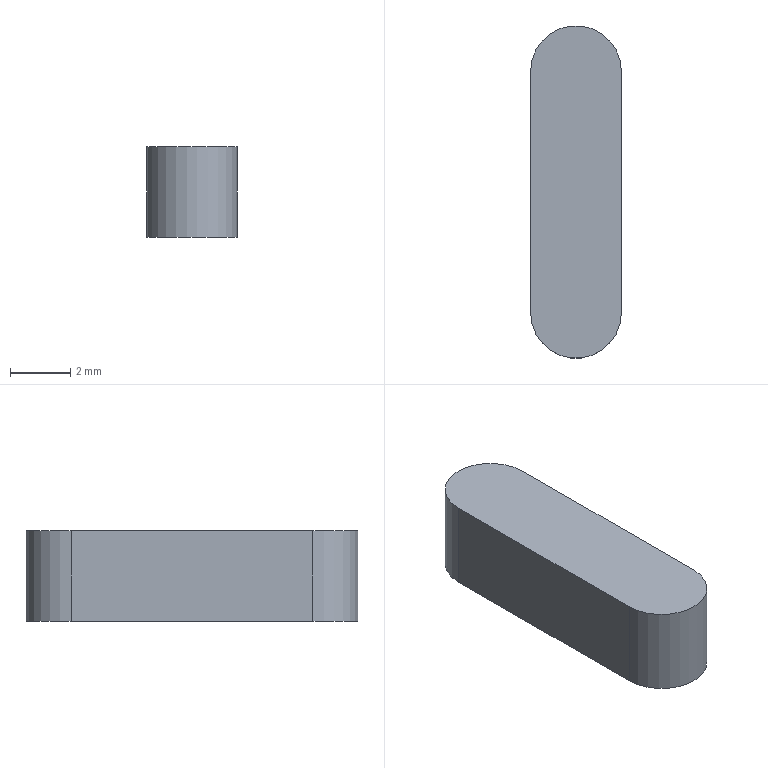Component | NX | FLAT_KEY | 1 solid | 6 faces | box 3 x 11 x 3 mm | volume 93 mm3 | plane 4 | cylinder 2 | commonest cylinder face diameters 3 x2
STEP:
#1=CARTESIAN_POINT('',(0.,0.,0.));
#2=DIRECTION('',(0.,0.,1.));
#3=DIRECTION('',(1.,0.,0.));
#4=AXIS2_PLACEMENT_3D('',#1,#2,#3);
#5=CARTESIAN_POINT('',(1.5,76.,92.25));
#6=VERTEX_POINT('',#5);
#7=CARTESIAN_POINT('',(1.5,68.,92.25));
#8=VERTEX_POINT('',#7);
#9=CARTESIAN_POINT('',(1.5,72.,92.25));
#10=DIRECTION('',(0.,-1.,0.));
#11=VECTOR('',#10,1.);
#12=LINE('',#9,#11);
#13=CARTESIAN_POINT('',(0.,72.,92.25));
#14=DIRECTION('',(0.,0.,1.));
#15=DIRECTION('',(0.,1.,0.));
#16=AXIS2_PLACEMENT_3D('',#13,#14,#15);
#17=PLANE('',#16);
#18=CARTESIAN_POINT('',(0.,-1.5));
#19=DIRECTION('',(-1.,0.));
#20=VECTOR('',#19,1.);
#21=LINE('',#18,#20);
#22=(GEOMETRIC_REPRESENTATION_CONTEXT(2)PARAMETRIC_REPRESENTATION_CONTEXT()REPRESENTATION_CONTEXT('',''));
#23=DEFINITIONAL_REPRESENTATION('',(#21),#22);
#24=PCURVE('',#17,#23);
#25=CARTESIAN_POINT('',(1.5,72.,89.25));
#26=DIRECTION('',(1.,0.,0.));
#27=DIRECTION('',(0.,0.,-1.));
#28=AXIS2_PLACEMENT_3D('',#25,#26,#27);
#29=PLANE('',#28);
#30=CARTESIAN_POINT('',(-3.,0.));
#31=DIRECTION('',(0.,-1.));
#32=VECTOR('',#31,1.);
#33=LINE('',#30,#32);
#34=(GEOMETRIC_REPRESENTATION_CONTEXT(2)PARAMETRIC_REPRESENTATION_CONTEXT()REPRESENTATION_CONTEXT('',''));
#35=DEFINITIONAL_REPRESENTATION('',(#33),#34);
#36=PCURVE('',#29,#35);
#37=SURFACE_CURVE('',#12,(#24,#36),.PCURVE_S1.);
#38=EDGE_CURVE('',#6,#8,#37,.T.);
#39=ORIENTED_EDGE('',*,*,#38,.F.);
#40=CARTESIAN_POINT('',(-1.5,76.,92.25));
#41=VERTEX_POINT('',#40);
#42=CARTESIAN_POINT('',(0.,76.,92.25));
#43=DIRECTION('',(0.,0.,1.));
#44=DIRECTION('',(0.,1.,0.));
#45=AXIS2_PLACEMENT_3D('',#42,#43,#44);
#46=CIRCLE('',#45,1.5);
#47=CARTESIAN_POINT('',(4.,0.));
#48=DIRECTION('',(1.,0.));
#49=AXIS2_PLACEMENT_2D('',#47,#48);
#50=CIRCLE('',#49,1.5);
#51=(GEOMETRIC_REPRESENTATION_CONTEXT(2)PARAMETRIC_REPRESENTATION_CONTEXT()REPRESENTATION_CONTEXT('',''));
#52=DEFINITIONAL_REPRESENTATION('',(#50),#51);
#53=PCURVE('',#17,#52);
#54=CARTESIAN_POINT('',(0.,76.,89.25));
#55=DIRECTION('',(0.,0.,1.));
#56=DIRECTION('',(0.,1.,0.));
#57=AXIS2_PLACEMENT_3D('',#54,#55,#56);
#58=CYLINDRICAL_SURFACE('',#57,1.5);
#59=CARTESIAN_POINT('',(0.,3.));
#60=DIRECTION('',(1.,0.));
#61=VECTOR('',#60,1.);
#62=LINE('',#59,#61);
#63=(GEOMETRIC_REPRESENTATION_CONTEXT(2)PARAMETRIC_REPRESENTATION_CONTEXT()REPRESENTATION_CONTEXT('',''));
#64=DEFINITIONAL_REPRESENTATION('',(#62),#63);
#65=PCURVE('',#58,#64);
#66=SURFACE_CURVE('',#46,(#53,#65),.PCURVE_S1.);
#67=EDGE_CURVE('',#6,#41,#66,.T.);
#68=ORIENTED_EDGE('',*,*,#67,.T.);
#69=CARTESIAN_POINT('',(-1.5,68.,92.25));
#70=VERTEX_POINT('',#69);
#71=CARTESIAN_POINT('',(-1.5,72.,92.25));
#72=DIRECTION('',(0.,1.,0.));
#73=VECTOR('',#72,1.);
#74=LINE('',#71,#73);
#75=CARTESIAN_POINT('',(0.,1.5));
#76=DIRECTION('',(1.,0.));
#77=VECTOR('',#76,1.);
#78=LINE('',#75,#77);
#79=(GEOMETRIC_REPRESENTATION_CONTEXT(2)PARAMETRIC_REPRESENTATION_CONTEXT()REPRESENTATION_CONTEXT('',''));
#80=DEFINITIONAL_REPRESENTATION('',(#78),#79);
#81=PCURVE('',#17,#80);
#82=CARTESIAN_POINT('',(-1.5,72.,89.25));
#83=DIRECTION('',(-1.,0.,0.));
#84=DIRECTION('',(0.,0.,1.));
#85=AXIS2_PLACEMENT_3D('',#82,#83,#84);
#86=PLANE('',#85);
#87=CARTESIAN_POINT('',(3.,0.));
#88=DIRECTION('',(0.,1.));
#89=VECTOR('',#88,1.);
#90=LINE('',#87,#89);
#91=(GEOMETRIC_REPRESENTATION_CONTEXT(2)PARAMETRIC_REPRESENTATION_CONTEXT()REPRESENTATION_CONTEXT('',''));
#92=DEFINITIONAL_REPRESENTATION('',(#90),#91);
#93=PCURVE('',#86,#92);
#94=SURFACE_CURVE('',#74,(#81,#93),.PCURVE_S1.);
#95=EDGE_CURVE('',#70,#41,#94,.T.);
#96=ORIENTED_EDGE('',*,*,#95,.F.);
#97=CARTESIAN_POINT('',(0.,68.,92.25));
#98=DIRECTION('',(0.,0.,1.));
#99=DIRECTION('',(0.,1.,0.));
#100=AXIS2_PLACEMENT_3D('',#97,#98,#99);
#101=CIRCLE('',#100,1.5);
#102=CARTESIAN_POINT('',(-4.,0.));
#103=DIRECTION('',(1.,0.));
#104=AXIS2_PLACEMENT_2D('',#102,#103);
#105=CIRCLE('',#104,1.5);
#106=(GEOMETRIC_REPRESENTATION_CONTEXT(2)PARAMETRIC_REPRESENTATION_CONTEXT()REPRESENTATION_CONTEXT('',''));
#107=DEFINITIONAL_REPRESENTATION('',(#105),#106);
#108=PCURVE('',#17,#107);
#109=CARTESIAN_POINT('',(0.,68.,89.25));
#110=DIRECTION('',(0.,0.,1.));
#111=DIRECTION('',(0.,1.,0.));
#112=AXIS2_PLACEMENT_3D('',#109,#110,#111);
#113=CYLINDRICAL_SURFACE('',#112,1.5);
#114=CARTESIAN_POINT('',(0.,3.));
#115=DIRECTION('',(1.,0.));
#116=VECTOR('',#115,1.);
#117=LINE('',#114,#116);
#118=(GEOMETRIC_REPRESENTATION_CONTEXT(2)PARAMETRIC_REPRESENTATION_CONTEXT()REPRESENTATION_CONTEXT('',''));
#119=DEFINITIONAL_REPRESENTATION('',(#117),#118);
#120=PCURVE('',#113,#119);
#121=SURFACE_CURVE('',#101,(#108,#120),.PCURVE_S1.);
#122=EDGE_CURVE('',#70,#8,#121,.T.);
#123=ORIENTED_EDGE('',*,*,#122,.T.);
#124=EDGE_LOOP('',(#39,#68,#96,#123));
#125=FACE_BOUND('',#124,.T.);
#126=ADVANCED_FACE('',(#125),#17,.T.);
#127=CARTESIAN_POINT('',(1.5,68.,89.25));
#128=VERTEX_POINT('',#127);
#129=CARTESIAN_POINT('',(1.5,76.,89.25));
#130=VERTEX_POINT('',#129);
#131=CARTESIAN_POINT('',(1.5,72.,89.25));
#132=DIRECTION('',(0.,1.,0.));
#133=VECTOR('',#132,1.);
#134=LINE('',#131,#133);
#135=CARTESIAN_POINT('',(0.,0.));
#136=DIRECTION('',(0.,1.));
#137=VECTOR('',#136,1.);
#138=LINE('',#135,#137);
#139=(GEOMETRIC_REPRESENTATION_CONTEXT(2)PARAMETRIC_REPRESENTATION_CONTEXT()REPRESENTATION_CONTEXT('',''));
#140=DEFINITIONAL_REPRESENTATION('',(#138),#139);
#141=PCURVE('',#29,#140);
#142=CARTESIAN_POINT('',(0.,72.,89.25));
#143=DIRECTION('',(0.,0.,-1.));
#144=DIRECTION('',(0.,-1.,0.));
#145=AXIS2_PLACEMENT_3D('',#142,#143,#144);
#146=PLANE('',#145);
#147=CARTESIAN_POINT('',(0.,-1.5));
#148=DIRECTION('',(-1.,0.));
#149=VECTOR('',#148,1.);
#150=LINE('',#147,#149);
#151=(GEOMETRIC_REPRESENTATION_CONTEXT(2)PARAMETRIC_REPRESENTATION_CONTEXT()REPRESENTATION_CONTEXT('',''));
#152=DEFINITIONAL_REPRESENTATION('',(#150),#151);
#153=PCURVE('',#146,#152);
#154=SURFACE_CURVE('',#134,(#141,#153),.PCURVE_S1.);
#155=EDGE_CURVE('',#128,#130,#154,.T.);
#156=ORIENTED_EDGE('',*,*,#155,.T.);
#157=CARTESIAN_POINT('',(1.5,76.,89.25));
#158=DIRECTION('',(0.,0.,1.));
#159=VECTOR('',#158,1.);
#160=LINE('',#157,#159);
#161=CARTESIAN_POINT('',(0.,4.));
#162=DIRECTION('',(-1.,0.));
#163=VECTOR('',#162,1.);
#164=LINE('',#161,#163);
#165=(GEOMETRIC_REPRESENTATION_CONTEXT(2)PARAMETRIC_REPRESENTATION_CONTEXT()REPRESENTATION_CONTEXT('',''));
#166=DEFINITIONAL_REPRESENTATION('',(#164),#165);
#167=PCURVE('',#29,#166);
#168=CARTESIAN_POINT('',(4.712,0.));
#169=DIRECTION('',(0.,1.));
#170=VECTOR('',#169,1.);
#171=LINE('',#168,#170);
#172=(GEOMETRIC_REPRESENTATION_CONTEXT(2)PARAMETRIC_REPRESENTATION_CONTEXT()REPRESENTATION_CONTEXT('',''));
#173=DEFINITIONAL_REPRESENTATION('',(#171),#172);
#174=PCURVE('',#58,#173);
#175=SURFACE_CURVE('',#160,(#167,#174),.PCURVE_S1.);
#176=EDGE_CURVE('',#130,#6,#175,.T.);
#177=ORIENTED_EDGE('',*,*,#176,.T.);
#178=ORIENTED_EDGE('',*,*,#38,.T.);
#179=CARTESIAN_POINT('',(1.5,68.,89.25));
#180=DIRECTION('',(0.,0.,-1.));
#181=VECTOR('',#180,1.);
#182=LINE('',#179,#181);
#183=CARTESIAN_POINT('',(0.,-4.));
#184=DIRECTION('',(1.,0.));
#185=VECTOR('',#184,1.);
#186=LINE('',#183,#185);
#187=(GEOMETRIC_REPRESENTATION_CONTEXT(2)PARAMETRIC_REPRESENTATION_CONTEXT()REPRESENTATION_CONTEXT('',''));
#188=DEFINITIONAL_REPRESENTATION('',(#186),#187);
#189=PCURVE('',#29,#188);
#190=CARTESIAN_POINT('',(4.712,0.));
#191=DIRECTION('',(0.,-1.));
#192=VECTOR('',#191,1.);
#193=LINE('',#190,#192);
#194=(GEOMETRIC_REPRESENTATION_CONTEXT(2)PARAMETRIC_REPRESENTATION_CONTEXT()REPRESENTATION_CONTEXT('',''));
#195=DEFINITIONAL_REPRESENTATION('',(#193),#194);
#196=PCURVE('',#113,#195);
#197=SURFACE_CURVE('',#182,(#189,#196),.PCURVE_S1.);
#198=EDGE_CURVE('',#8,#128,#197,.T.);
#199=ORIENTED_EDGE('',*,*,#198,.T.);
#200=EDGE_LOOP('',(#156,#177,#178,#199));
#201=FACE_BOUND('',#200,.T.);
#202=ADVANCED_FACE('',(#201),#29,.T.);
#203=ORIENTED_EDGE('',*,*,#95,.T.);
#204=CARTESIAN_POINT('',(-1.5,76.,89.25));
#205=VERTEX_POINT('',#204);
#206=CARTESIAN_POINT('',(-1.5,76.,89.25));
#207=DIRECTION('',(0.,0.,-1.));
#208=VECTOR('',#207,1.);
#209=LINE('',#206,#208);
#210=CARTESIAN_POINT('',(0.,4.));
#211=DIRECTION('',(-1.,0.));
#212=VECTOR('',#211,1.);
#213=LINE('',#210,#212);
#214=(GEOMETRIC_REPRESENTATION_CONTEXT(2)PARAMETRIC_REPRESENTATION_CONTEXT()REPRESENTATION_CONTEXT('',''));
#215=DEFINITIONAL_REPRESENTATION('',(#213),#214);
#216=PCURVE('',#86,#215);
#217=CARTESIAN_POINT('',(7.854,0.));
#218=DIRECTION('',(0.,-1.));
#219=VECTOR('',#218,1.);
#220=LINE('',#217,#219);
#221=(GEOMETRIC_REPRESENTATION_CONTEXT(2)PARAMETRIC_REPRESENTATION_CONTEXT()REPRESENTATION_CONTEXT('',''));
#222=DEFINITIONAL_REPRESENTATION('',(#220),#221);
#223=PCURVE('',#58,#222);
#224=SURFACE_CURVE('',#209,(#216,#223),.PCURVE_S1.);
#225=EDGE_CURVE('',#41,#205,#224,.T.);
#226=ORIENTED_EDGE('',*,*,#225,.T.);
#227=CARTESIAN_POINT('',(-1.5,68.,89.25));
#228=VERTEX_POINT('',#227);
#229=CARTESIAN_POINT('',(-1.5,72.,89.25));
#230=DIRECTION('',(0.,-1.,0.));
#231=VECTOR('',#230,1.);
#232=LINE('',#229,#231);
#233=CARTESIAN_POINT('',(0.,0.));
#234=DIRECTION('',(0.,-1.));
#235=VECTOR('',#234,1.);
#236=LINE('',#233,#235);
#237=(GEOMETRIC_REPRESENTATION_CONTEXT(2)PARAMETRIC_REPRESENTATION_CONTEXT()REPRESENTATION_CONTEXT('',''));
#238=DEFINITIONAL_REPRESENTATION('',(#236),#237);
#239=PCURVE('',#86,#238);
#240=CARTESIAN_POINT('',(0.,1.5));
#241=DIRECTION('',(1.,0.));
#242=VECTOR('',#241,1.);
#243=LINE('',#240,#242);
#244=(GEOMETRIC_REPRESENTATION_CONTEXT(2)PARAMETRIC_REPRESENTATION_CONTEXT()REPRESENTATION_CONTEXT('',''));
#245=DEFINITIONAL_REPRESENTATION('',(#243),#244);
#246=PCURVE('',#146,#245);
#247=SURFACE_CURVE('',#232,(#239,#246),.PCURVE_S1.);
#248=EDGE_CURVE('',#205,#228,#247,.T.);
#249=ORIENTED_EDGE('',*,*,#248,.T.);
#250=CARTESIAN_POINT('',(-1.5,68.,89.25));
#251=DIRECTION('',(0.,0.,1.));
#252=VECTOR('',#251,1.);
#253=LINE('',#250,#252);
#254=CARTESIAN_POINT('',(0.,-4.));
#255=DIRECTION('',(1.,0.));
#256=VECTOR('',#255,1.);
#257=LINE('',#254,#256);
#258=(GEOMETRIC_REPRESENTATION_CONTEXT(2)PARAMETRIC_REPRESENTATION_CONTEXT()REPRESENTATION_CONTEXT('',''));
#259=DEFINITIONAL_REPRESENTATION('',(#257),#258);
#260=PCURVE('',#86,#259);
#261=CARTESIAN_POINT('',(1.571,0.));
#262=DIRECTION('',(0.,1.));
#263=VECTOR('',#262,1.);
#264=LINE('',#261,#263);
#265=(GEOMETRIC_REPRESENTATION_CONTEXT(2)PARAMETRIC_REPRESENTATION_CONTEXT()REPRESENTATION_CONTEXT('',''));
#266=DEFINITIONAL_REPRESENTATION('',(#264),#265);
#267=PCURVE('',#113,#266);
#268=SURFACE_CURVE('',#253,(#260,#267),.PCURVE_S1.);
#269=EDGE_CURVE('',#228,#70,#268,.T.);
#270=ORIENTED_EDGE('',*,*,#269,.T.);
#271=EDGE_LOOP('',(#203,#226,#249,#270));
#272=FACE_BOUND('',#271,.T.);
#273=ADVANCED_FACE('',(#272),#86,.T.);
#274=CARTESIAN_POINT('',(0.,76.,89.25));
#275=DIRECTION('',(0.,0.,-1.));
#276=DIRECTION('',(0.,-1.,0.));
#277=AXIS2_PLACEMENT_3D('',#274,#275,#276);
#278=CIRCLE('',#277,1.5);
#279=CARTESIAN_POINT('',(-4.,0.));
#280=DIRECTION('',(1.,0.));
#281=AXIS2_PLACEMENT_2D('',#279,#280);
#282=CIRCLE('',#281,1.5);
#283=(GEOMETRIC_REPRESENTATION_CONTEXT(2)PARAMETRIC_REPRESENTATION_CONTEXT()REPRESENTATION_CONTEXT('',''));
#284=DEFINITIONAL_REPRESENTATION('',(#282),#283);
#285=PCURVE('',#146,#284);
#286=CARTESIAN_POINT('',(9.425,0.));
#287=DIRECTION('',(-1.,0.));
#288=VECTOR('',#287,1.);
#289=LINE('',#286,#288);
#290=(GEOMETRIC_REPRESENTATION_CONTEXT(2)PARAMETRIC_REPRESENTATION_CONTEXT()REPRESENTATION_CONTEXT('',''));
#291=DEFINITIONAL_REPRESENTATION('',(#289),#290);
#292=PCURVE('',#58,#291);
#293=SURFACE_CURVE('',#278,(#285,#292),.PCURVE_S1.);
#294=EDGE_CURVE('',#205,#130,#293,.T.);
#295=ORIENTED_EDGE('',*,*,#294,.T.);
#296=ORIENTED_EDGE('',*,*,#155,.F.);
#297=CARTESIAN_POINT('',(0.,68.,89.25));
#298=DIRECTION('',(0.,0.,-1.));
#299=DIRECTION('',(0.,-1.,0.));
#300=AXIS2_PLACEMENT_3D('',#297,#298,#299);
#301=CIRCLE('',#300,1.5);
#302=CARTESIAN_POINT('',(4.,0.));
#303=DIRECTION('',(1.,0.));
#304=AXIS2_PLACEMENT_2D('',#302,#303);
#305=CIRCLE('',#304,1.5);
#306=(GEOMETRIC_REPRESENTATION_CONTEXT(2)PARAMETRIC_REPRESENTATION_CONTEXT()REPRESENTATION_CONTEXT('',''));
#307=DEFINITIONAL_REPRESENTATION('',(#305),#306);
#308=PCURVE('',#146,#307);
#309=CARTESIAN_POINT('',(9.425,0.));
#310=DIRECTION('',(-1.,0.));
#311=VECTOR('',#310,1.);
#312=LINE('',#309,#311);
#313=(GEOMETRIC_REPRESENTATION_CONTEXT(2)PARAMETRIC_REPRESENTATION_CONTEXT()REPRESENTATION_CONTEXT('',''));
#314=DEFINITIONAL_REPRESENTATION('',(#312),#313);
#315=PCURVE('',#113,#314);
#316=SURFACE_CURVE('',#301,(#308,#315),.PCURVE_S1.);
#317=EDGE_CURVE('',#128,#228,#316,.T.);
#318=ORIENTED_EDGE('',*,*,#317,.T.);
#319=ORIENTED_EDGE('',*,*,#248,.F.);
#320=EDGE_LOOP('',(#295,#296,#318,#319));
#321=FACE_BOUND('',#320,.T.);
#322=ADVANCED_FACE('',(#321),#146,.T.);
#323=ORIENTED_EDGE('',*,*,#67,.F.);
#324=ORIENTED_EDGE('',*,*,#176,.F.);
#325=ORIENTED_EDGE('',*,*,#294,.F.);
#326=ORIENTED_EDGE('',*,*,#225,.F.);
#327=EDGE_LOOP('',(#323,#324,#325,#326));
#328=FACE_BOUND('',#327,.T.);
#329=ADVANCED_FACE('',(#328),#58,.T.);
#330=ORIENTED_EDGE('',*,*,#269,.F.);
#331=ORIENTED_EDGE('',*,*,#317,.F.);
#332=ORIENTED_EDGE('',*,*,#198,.F.);
#333=ORIENTED_EDGE('',*,*,#122,.F.);
#334=EDGE_LOOP('',(#330,#331,#332,#333));
#335=FACE_BOUND('',#334,.T.);
#336=ADVANCED_FACE('',(#335),#113,.T.);
#337=CLOSED_SHELL('',(#126,#202,#273,#322,#329,#336));
#338=MANIFOLD_SOLID_BREP('',#337);
#339=(LENGTH_UNIT()NAMED_UNIT(*)SI_UNIT(.MILLI.,.METRE.));
#340=UNCERTAINTY_MEASURE_WITH_UNIT(LENGTH_MEASURE(0.0000001),#339,'','');
#341=(NAMED_UNIT(*)PLANE_ANGLE_UNIT()SI_UNIT($,.RADIAN.));
#342=(NAMED_UNIT(*)SI_UNIT($,.STERADIAN.)SOLID_ANGLE_UNIT());
#343=(GEOMETRIC_REPRESENTATION_CONTEXT(3)GLOBAL_UNCERTAINTY_ASSIGNED_CONTEXT((#340))GLOBAL_UNIT_ASSIGNED_CONTEXT((#339,#341,#342))REPRESENTATION_CONTEXT('',''));
#344=ADVANCED_BREP_SHAPE_REPRESENTATION('',(#4,#338),#343);